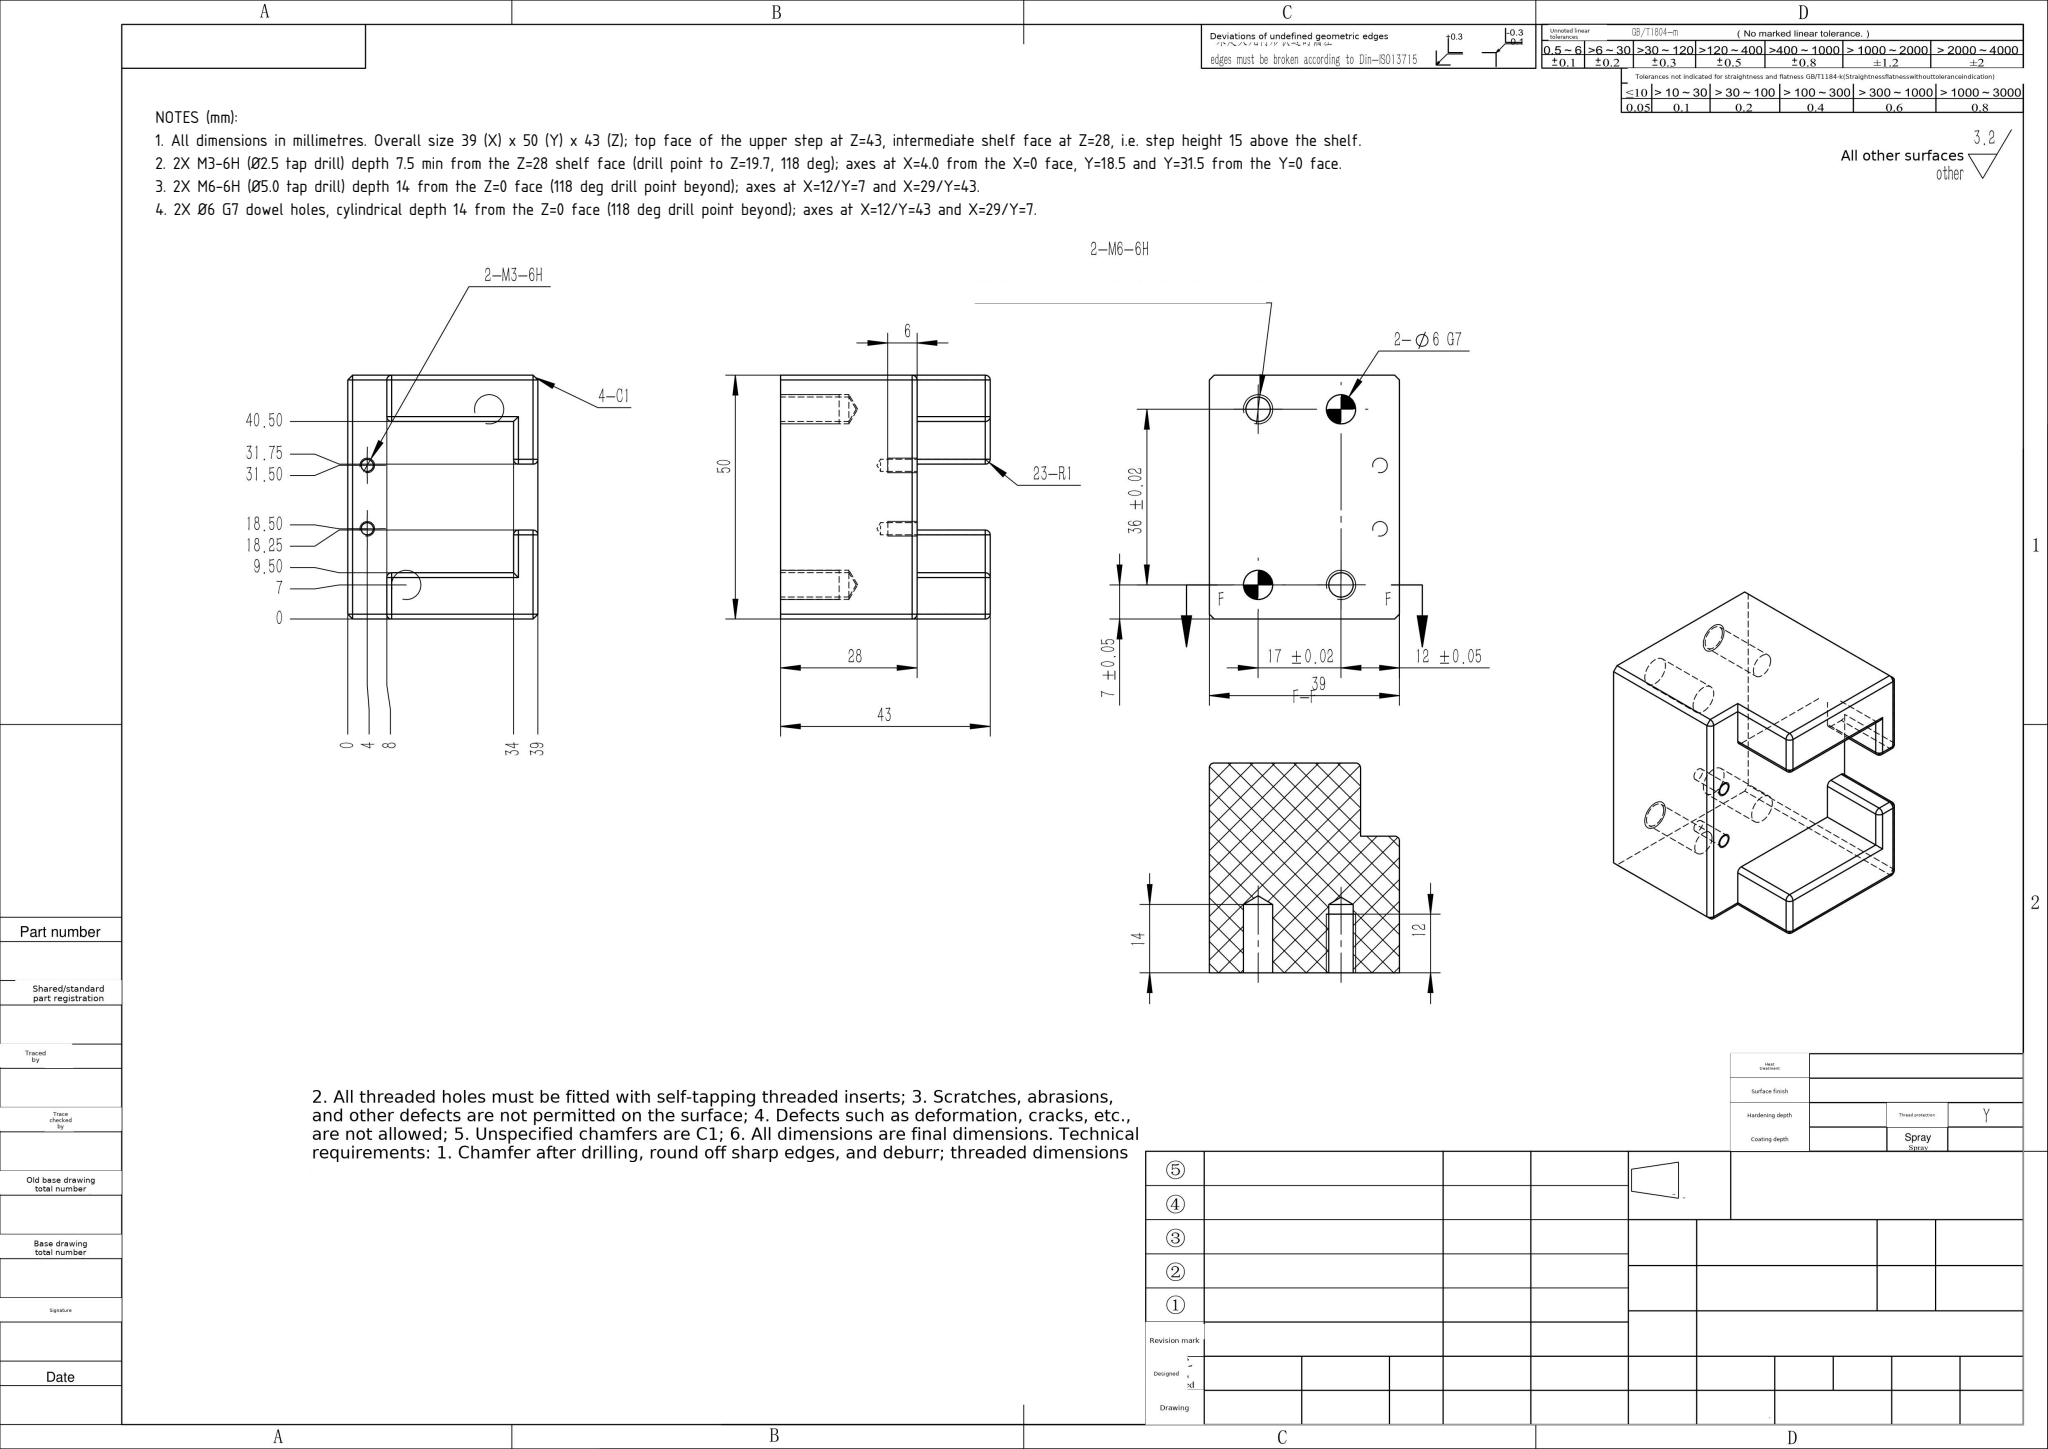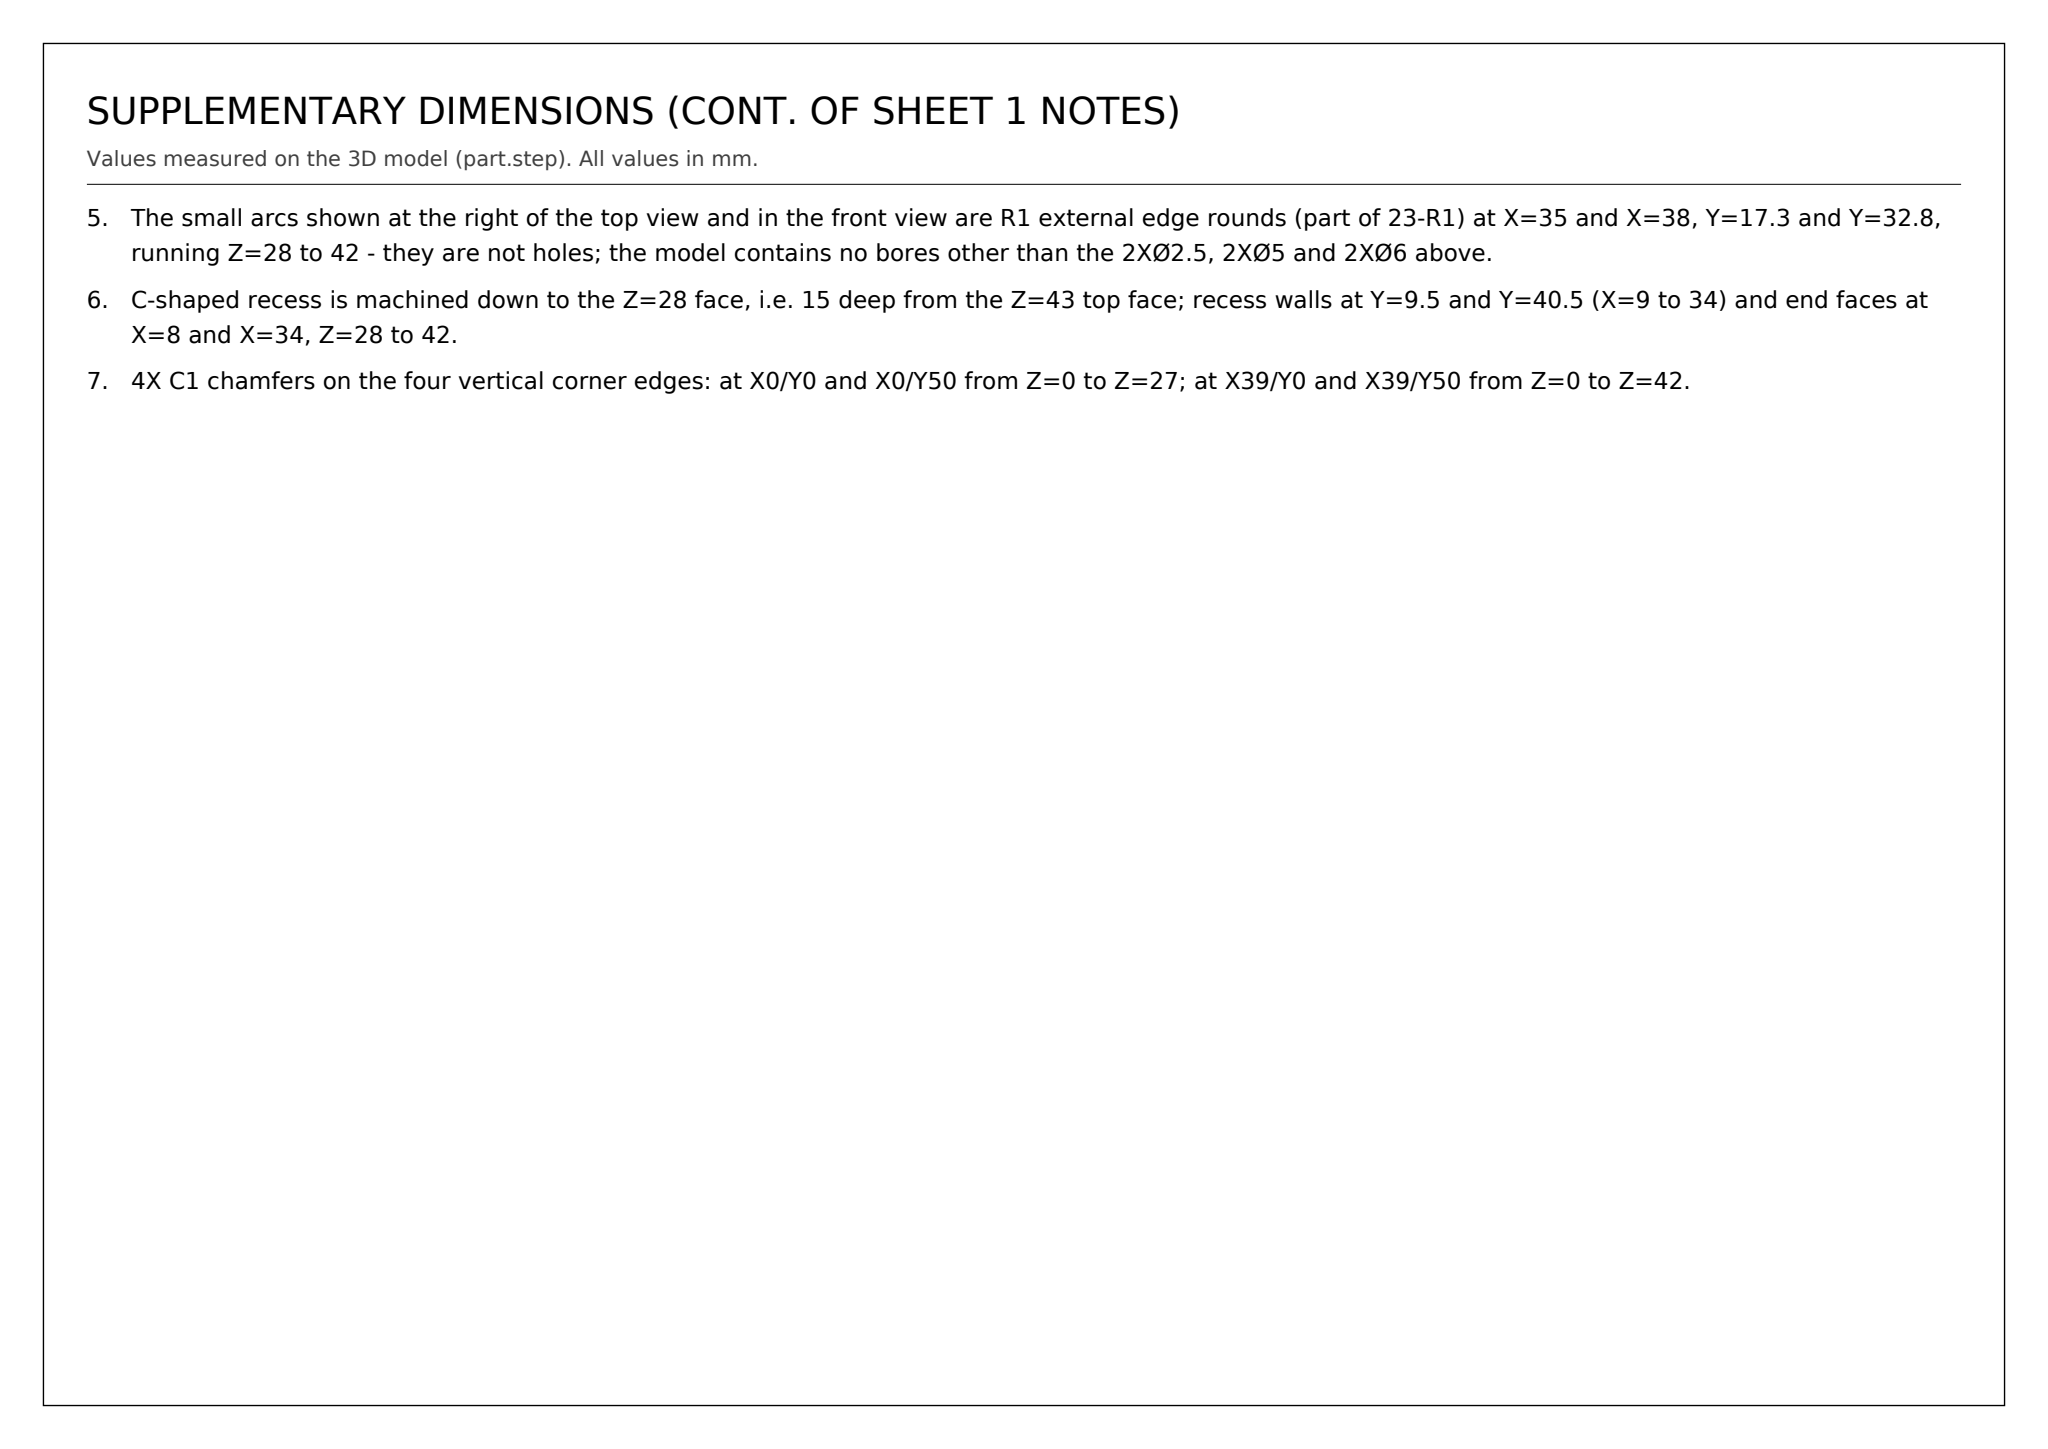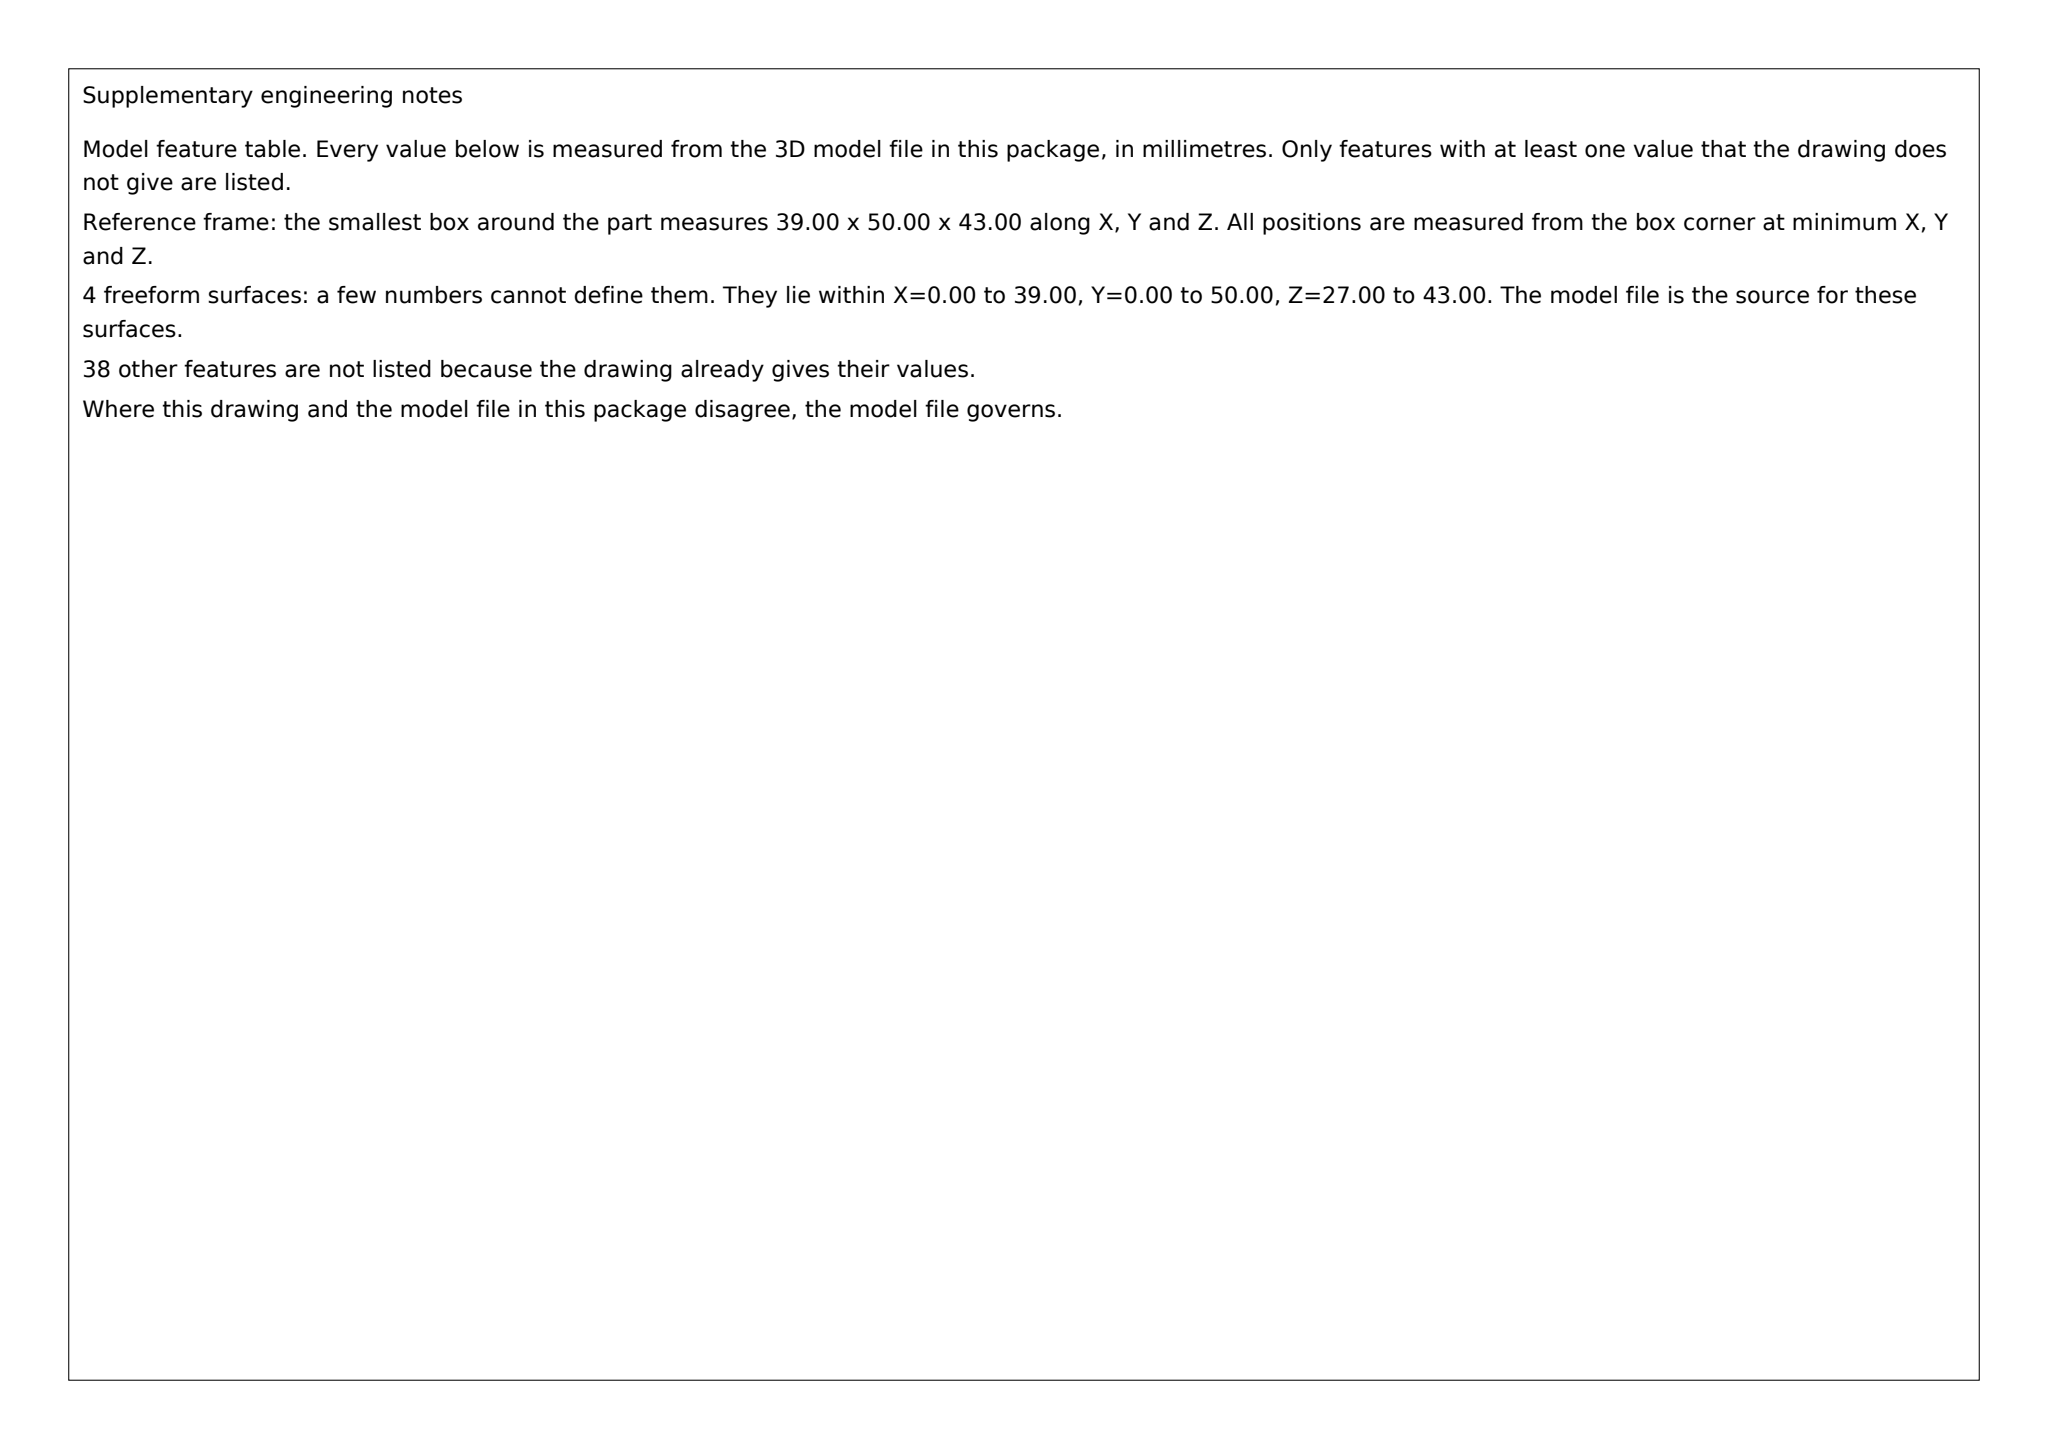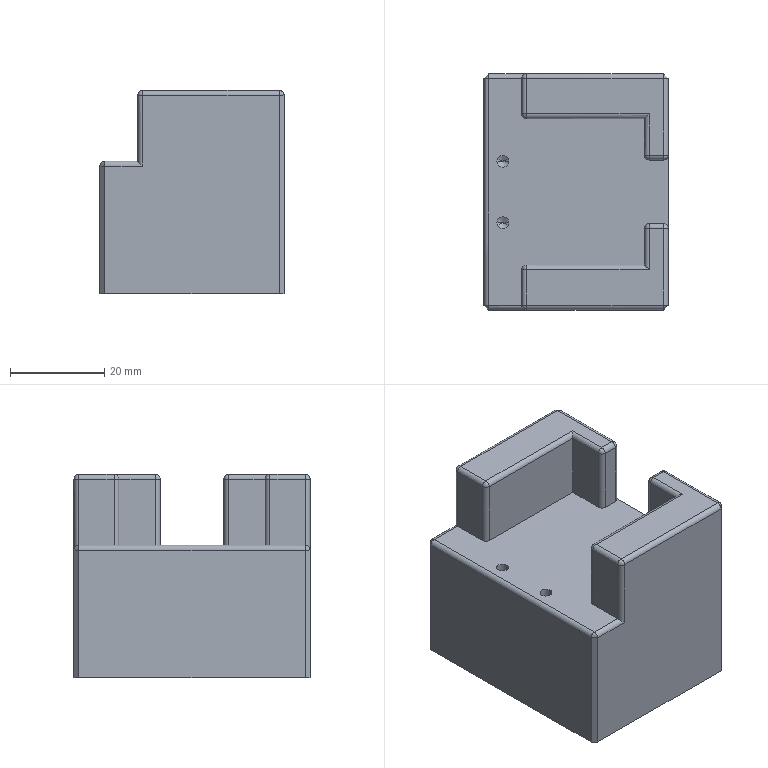Part | SolidWorks | mm | 1 solid | 79 faces | box 39 x 50 x 43 mm | volume 63125 mm3 | cylinder 35 | plane 20 | cone 12 | sphere 8 | spline 4 | commonest cylinder face diameters 2 x23 2.5 x4 6 x4 5 x4
Drawing notes:
All dimensions in millimetres. Overall size 39 (X) x 50 (Y) x 43 (Z); top face of the upper step at Z=43, intermediate shelf face at Z=28, i.e. step height 15 above the shelf. | from the solid: bbox_xyz [39.0,50.0,43.0]; axis_planes z=0, z=28 (x1-39, y1-49) and z=43 (x9-38)
2X M3-6H (Ø2.5 tap drill) depth 7.5 min from the Z=28 shelf face (drill point to Z=19.7, 118 deg); axes at X=4.0 from the X=0 face, Y=18.5 and Y=31.5 from the Y=0 face. | from the solid: cylinders hole/bore dia 2.5, axis z at (4.0,18.5) and (4.0,31.5), from 20.5 to 28; cones 118 deg ref_dia 2.5 at z 19.7-20.5
2X M6-6H (Ø5.0 tap drill) depth 14 from the Z=0 face (118 deg drill point beyond); axes at X=12/Y=7 and X=29/Y=43. | from the solid: cylinders hole/bore dia 5.0, axis z at (12,7) and (29,43), from 0.0 to 14.0; cones 118 deg ref_dia 5.0 at z=14
2X Ø6 G7 dowel holes, cylindrical depth 14 from the Z=0 face (118 deg drill point beyond); axes at X=12/Y=43 and X=29/Y=7. | from the solid: cylinders hole/bore dia 6.0, axis z at (12,43) and (29,7), from 0.0 to 14.0; cones 118 deg ref_dia 6.0 at z=14
The small arcs shown at the right of the top view and in the front view are R1 external edge rounds (part of 23-R1) at X=35 and X=38, Y=17.3 and Y=32.8, running Z=28 to 42 - they are not holes; the model contains no bores other than the 2XØ2.5, 2XØ5 and 2XØ6 above. | from the solid: convex arc (round/outer radius) dia 2.0 axis z at (35,17.3),(35,32.8),(38,17.3),(38,32.8) from z 28 to 42; cylinders list contains only six hole/bore entries
C-shaped recess is machined down to the Z=28 face, i.e. 15 deep from the Z=43 top face; recess walls at Y=9.5 and Y=40.5 (X=9 to 34) and end faces at X=8 and X=34, Z=28 to 42. | from the solid: axis_planes z=28 extent x[1,39] y[1,49]; y=9.5 and y=40.5 extent x[9,34] z[28,42]; x=34 extent y[9.5,17.3] and y[32.8,40.5] z[28,42]; x=8 extent y[1,8.5] and y[41.5,49] z[28,42]
4X C1 chamfers on the four vertical corner edges: at X0/Y0 and X0/Y50 from Z=0 to Z=27; at X39/Y0 and X39/Y50 from Z=0 to Z=42. | from the solid: inclined_planes 45/45/90 at bbox_from [0,0,0] and [0,49,0] size 1x1x27; at [38,0,0] and [38,49,0] size 1x1x42